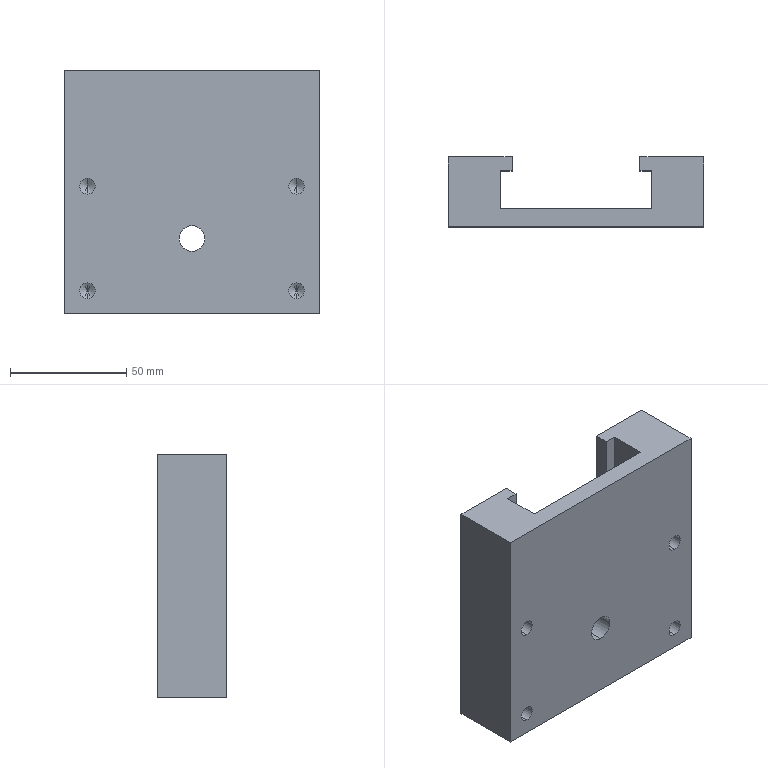Component | SolidWorks | BrassGuideRail-3 | 1 solid | 40 faces | box 110 x 30 x 105 mm | volume 198159 mm3 | cylinder 14 | plane 14 | cone 12 | commonest cylinder face diameters 6.8 x8 4.2 x4 11 x2
build123d program:
from build123d import *

# Parameters (mm, degrees)
EXTRUDE1_DEPTH        = 105
SKETCH2_R             = 5.5
EXTRUDE2_DEPTH        = 105
M5_TAPPED_HOLE1_D     = 4.2
M5_TAPPED_HOLE1_DEPTH = 14
M5_TAPPED_HOLE1_TIP   = 1.262
M8_TAPPED_HOLE2_D     = 6.8
M8_TAPPED_HOLE2_DEPTH = 22.25
M8_TAPPED_HOLE2_TIP   = 2.043


with BuildPart() as part:
    # Sketch1 → Extrude1 (new body)
    with BuildSketch(Plane.XY):
        Polygon((-55, 15), (-27.5, 15), (-27.5, 9), (-32.5, 9), (-32.5, -7), (32.5, -7), (32.5, 9), (27.5, 9), (27.5, 15), (55, 15), (55, -15), (-55, -15), align=None)
    extrude(amount=EXTRUDE1_DEPTH)

    # Sketch2 → Extrude2 (cut)
    with BuildSketch(Plane(origin=(0, -7, 0), x_dir=(1, 0, 0), z_dir=(0, 1, 0))):
        with Locations(Location((0, -32.5, 0), (0, 0, 270))):
            Circle(SKETCH2_R)
    extrude(amount=-EXTRUDE2_DEPTH, mode=Mode.SUBTRACT)

    # M5 Tapped Hole1
    with Locations(Plane(origin=(0, 15, 0), x_dir=(-1, 0, 0), z_dir=(0, 1, 0))):
        with Locations((45, 85), (-45, 85)):
            Hole(M5_TAPPED_HOLE1_D / 2, depth=M5_TAPPED_HOLE1_DEPTH)
            with Locations((0, 0, -(M5_TAPPED_HOLE1_DEPTH + M5_TAPPED_HOLE1_TIP / 2))):  # 118° drill point
                Cone(0, M5_TAPPED_HOLE1_D / 2, M5_TAPPED_HOLE1_TIP, mode=Mode.SUBTRACT)

    # M8 Tapped Hole2
    with Locations(Plane.XZ.offset(15)):
        with Locations((-45, 10), (45, 10), (45, 55), (-45, 55)):
            Hole(M8_TAPPED_HOLE2_D / 2, depth=M8_TAPPED_HOLE2_DEPTH)
            with Locations((0, 0, -(M8_TAPPED_HOLE2_DEPTH + M8_TAPPED_HOLE2_TIP / 2))):  # 118° drill point
                Cone(0, M8_TAPPED_HOLE2_D / 2, M8_TAPPED_HOLE2_TIP, mode=Mode.SUBTRACT)


solid = part.part

# Placed as in the assembly
solid = solid.moved(Location((250.216, 518.983, 27.106), (0, 0, 0)))
STEP:
#1=COLOUR_RGB('',0.7922,0.8196,0.9333);
#2=FILL_AREA_STYLE_COLOUR('',#1);
#3=FILL_AREA_STYLE('',(#2));
#4=SURFACE_STYLE_FILL_AREA(#3);
#5=SURFACE_SIDE_STYLE('',(#4));
#6=SURFACE_STYLE_USAGE(.BOTH.,#5);
#7=PRESENTATION_STYLE_ASSIGNMENT((#6));
#8=CARTESIAN_POINT('',(8.079,20.718,1.595));
#9=VERTEX_POINT('',#8);
#10=CARTESIAN_POINT('',(8.079,20.718,1.327));
#11=VERTEX_POINT('',#10);
#12=CARTESIAN_POINT('',(8.079,20.718,1.461));
#13=DIRECTION('',(0.,-1.,0.));
#14=DIRECTION('',(0.,0.,-1.));
#15=AXIS2_PLACEMENT_3D('',#12,#13,#14);
#16=CIRCLE('',#15,0.1339);
#17=EDGE_CURVE('',#9,#11,#16,.T.);
#18=ORIENTED_EDGE('',*,*,#17,.F.);
#19=CARTESIAN_POINT('',(8.079,19.842,1.595));
#20=VERTEX_POINT('',#19);
#21=CARTESIAN_POINT('',(8.079,19.842,1.595));
#22=DIRECTION('',(0.,-1.,0.));
#23=VECTOR('',#22,39.37);
#24=LINE('',#21,#23);
#25=EDGE_CURVE('',#9,#20,#24,.T.);
#26=ORIENTED_EDGE('',*,*,#25,.T.);
#27=CARTESIAN_POINT('',(8.079,19.842,1.327));
#28=VERTEX_POINT('',#27);
#29=CARTESIAN_POINT('',(8.079,19.842,1.461));
#30=DIRECTION('',(0.,-1.,0.));
#31=DIRECTION('',(0.,0.,-1.));
#32=AXIS2_PLACEMENT_3D('',#29,#30,#31);
#33=CIRCLE('',#32,0.1339);
#34=EDGE_CURVE('',#20,#28,#33,.T.);
#35=ORIENTED_EDGE('',*,*,#34,.T.);
#36=CARTESIAN_POINT('',(8.079,19.842,1.327));
#37=DIRECTION('',(0.,-1.,0.));
#38=VECTOR('',#37,39.37);
#39=LINE('',#36,#38);
#40=EDGE_CURVE('',#11,#28,#39,.T.);
#41=ORIENTED_EDGE('',*,*,#40,.F.);
#42=EDGE_LOOP('',(#18,#26,#35,#41));
#43=FACE_OUTER_BOUND('',#42,.T.);
#44=CARTESIAN_POINT('',(8.079,19.842,1.461));
#45=DIRECTION('',(0.,-1.,0.));
#46=DIRECTION('',(0.,0.,-1.));
#47=AXIS2_PLACEMENT_3D('',#44,#45,#46);
#48=CYLINDRICAL_SURFACE('',#47,0.1339);
#49=ADVANCED_FACE('',(#43),#48,.F.);
#50=CARTESIAN_POINT('',(8.079,20.798,1.461));
#51=VERTEX_POINT('',#50);
#52=CARTESIAN_POINT('',(8.079,20.718,1.327));
#53=DIRECTION('',(0.,-0.515,-0.8572));
#54=VECTOR('',#53,39.37);
#55=LINE('',#52,#54);
#56=EDGE_CURVE('',#51,#11,#55,.T.);
#57=ORIENTED_EDGE('',*,*,#56,.F.);
#58=CARTESIAN_POINT('',(8.079,20.718,1.595));
#59=DIRECTION('',(0.,-0.515,0.8572));
#60=VECTOR('',#59,39.37);
#61=LINE('',#58,#60);
#62=EDGE_CURVE('',#51,#9,#61,.T.);
#63=ORIENTED_EDGE('',*,*,#62,.T.);
#64=ORIENTED_EDGE('',*,*,#17,.T.);
#65=EDGE_LOOP('',(#57,#63,#64));
#66=FACE_OUTER_BOUND('',#65,.T.);
#67=CARTESIAN_POINT('',(8.079,20.718,1.461));
#68=DIRECTION('',(0.,-1.,0.));
#69=DIRECTION('',(0.,0.,-1.));
#70=AXIS2_PLACEMENT_3D('',#67,#68,#69);
#71=CONICAL_SURFACE('',#70,0.1339,1.03);
#72=ADVANCED_FACE('',(#66),#71,.F.);
#73=CARTESIAN_POINT('',(11.623,20.718,1.595));
#74=VERTEX_POINT('',#73);
#75=CARTESIAN_POINT('',(11.623,20.718,1.327));
#76=VERTEX_POINT('',#75);
#77=CARTESIAN_POINT('',(11.623,20.718,1.461));
#78=DIRECTION('',(0.,-1.,0.));
#79=DIRECTION('',(0.,0.,-1.));
#80=AXIS2_PLACEMENT_3D('',#77,#78,#79);
#81=CIRCLE('',#80,0.1339);
#82=EDGE_CURVE('',#74,#76,#81,.T.);
#83=ORIENTED_EDGE('',*,*,#82,.F.);
#84=CARTESIAN_POINT('',(11.623,19.842,1.595));
#85=VERTEX_POINT('',#84);
#86=CARTESIAN_POINT('',(11.623,19.842,1.595));
#87=DIRECTION('',(0.,-1.,0.));
#88=VECTOR('',#87,39.37);
#89=LINE('',#86,#88);
#90=EDGE_CURVE('',#74,#85,#89,.T.);
#91=ORIENTED_EDGE('',*,*,#90,.T.);
#92=CARTESIAN_POINT('',(11.623,19.842,1.327));
#93=VERTEX_POINT('',#92);
#94=CARTESIAN_POINT('',(11.623,19.842,1.461));
#95=DIRECTION('',(0.,-1.,0.));
#96=DIRECTION('',(0.,0.,-1.));
#97=AXIS2_PLACEMENT_3D('',#94,#95,#96);
#98=CIRCLE('',#97,0.1339);
#99=EDGE_CURVE('',#85,#93,#98,.T.);
#100=ORIENTED_EDGE('',*,*,#99,.T.);
#101=CARTESIAN_POINT('',(11.623,19.842,1.327));
#102=DIRECTION('',(0.,-1.,0.));
#103=VECTOR('',#102,39.37);
#104=LINE('',#101,#103);
#105=EDGE_CURVE('',#76,#93,#104,.T.);
#106=ORIENTED_EDGE('',*,*,#105,.F.);
#107=EDGE_LOOP('',(#83,#91,#100,#106));
#108=FACE_OUTER_BOUND('',#107,.T.);
#109=CARTESIAN_POINT('',(11.623,19.842,1.461));
#110=DIRECTION('',(0.,-1.,0.));
#111=DIRECTION('',(0.,0.,-1.));
#112=AXIS2_PLACEMENT_3D('',#109,#110,#111);
#113=CYLINDRICAL_SURFACE('',#112,0.1339);
#114=ADVANCED_FACE('',(#108),#113,.F.);
#115=CARTESIAN_POINT('',(11.623,20.798,1.461));
#116=VERTEX_POINT('',#115);
#117=CARTESIAN_POINT('',(11.623,20.718,1.327));
#118=DIRECTION('',(0.,-0.515,-0.8572));
#119=VECTOR('',#118,39.37);
#120=LINE('',#117,#119);
#121=EDGE_CURVE('',#116,#76,#120,.T.);
#122=ORIENTED_EDGE('',*,*,#121,.F.);
#123=CARTESIAN_POINT('',(11.623,20.718,1.595));
#124=DIRECTION('',(0.,-0.515,0.8572));
#125=VECTOR('',#124,39.37);
#126=LINE('',#123,#125);
#127=EDGE_CURVE('',#116,#74,#126,.T.);
#128=ORIENTED_EDGE('',*,*,#127,.T.);
#129=ORIENTED_EDGE('',*,*,#82,.T.);
#130=EDGE_LOOP('',(#122,#128,#129));
#131=FACE_OUTER_BOUND('',#130,.T.);
#132=CARTESIAN_POINT('',(11.623,20.718,1.461));
#133=DIRECTION('',(0.,-1.,0.));
#134=DIRECTION('',(0.,0.,-1.));
#135=AXIS2_PLACEMENT_3D('',#132,#133,#134);
#136=CONICAL_SURFACE('',#135,0.1339,1.03);
#137=ADVANCED_FACE('',(#131),#136,.F.);
#138=CARTESIAN_POINT('',(11.623,20.718,3.366));
#139=VERTEX_POINT('',#138);
#140=CARTESIAN_POINT('',(11.623,20.718,3.099));
#141=VERTEX_POINT('',#140);
#142=CARTESIAN_POINT('',(11.623,20.718,3.233));
#143=DIRECTION('',(0.,-1.,0.));
#144=DIRECTION('',(0.,0.,-1.));
#145=AXIS2_PLACEMENT_3D('',#142,#143,#144);
#146=CIRCLE('',#145,0.1339);
#147=EDGE_CURVE('',#139,#141,#146,.T.);
#148=ORIENTED_EDGE('',*,*,#147,.F.);
#149=CARTESIAN_POINT('',(11.623,19.842,3.366));
#150=VERTEX_POINT('',#149);
#151=CARTESIAN_POINT('',(11.623,19.842,3.366));
#152=DIRECTION('',(0.,-1.,0.));
#153=VECTOR('',#152,39.37);
#154=LINE('',#151,#153);
#155=EDGE_CURVE('',#139,#150,#154,.T.);
#156=ORIENTED_EDGE('',*,*,#155,.T.);
#157=CARTESIAN_POINT('',(11.623,19.842,3.099));
#158=VERTEX_POINT('',#157);
#159=CARTESIAN_POINT('',(11.623,19.842,3.233));
#160=DIRECTION('',(0.,-1.,0.));
#161=DIRECTION('',(0.,0.,-1.));
#162=AXIS2_PLACEMENT_3D('',#159,#160,#161);
#163=CIRCLE('',#162,0.1339);
#164=EDGE_CURVE('',#150,#158,#163,.T.);
#165=ORIENTED_EDGE('',*,*,#164,.T.);
#166=CARTESIAN_POINT('',(11.623,19.842,3.099));
#167=DIRECTION('',(0.,-1.,0.));
#168=VECTOR('',#167,39.37);
#169=LINE('',#166,#168);
#170=EDGE_CURVE('',#141,#158,#169,.T.);
#171=ORIENTED_EDGE('',*,*,#170,.F.);
#172=EDGE_LOOP('',(#148,#156,#165,#171));
#173=FACE_OUTER_BOUND('',#172,.T.);
#174=CARTESIAN_POINT('',(11.623,19.842,3.233));
#175=DIRECTION('',(0.,-1.,0.));
#176=DIRECTION('',(0.,0.,-1.));
#177=AXIS2_PLACEMENT_3D('',#174,#175,#176);
#178=CYLINDRICAL_SURFACE('',#177,0.1339);
#179=ADVANCED_FACE('',(#173),#178,.F.);
#180=CARTESIAN_POINT('',(11.623,20.798,3.233));
#181=VERTEX_POINT('',#180);
#182=CARTESIAN_POINT('',(11.623,20.718,3.099));
#183=DIRECTION('',(0.,-0.515,-0.8572));
#184=VECTOR('',#183,39.37);
#185=LINE('',#182,#184);
#186=EDGE_CURVE('',#181,#141,#185,.T.);
#187=ORIENTED_EDGE('',*,*,#186,.F.);
#188=CARTESIAN_POINT('',(11.623,20.718,3.366));
#189=DIRECTION('',(0.,-0.515,0.8572));
#190=VECTOR('',#189,39.37);
#191=LINE('',#188,#190);
#192=EDGE_CURVE('',#181,#139,#191,.T.);
#193=ORIENTED_EDGE('',*,*,#192,.T.);
#194=ORIENTED_EDGE('',*,*,#147,.T.);
#195=EDGE_LOOP('',(#187,#193,#194));
#196=FACE_OUTER_BOUND('',#195,.T.);
#197=CARTESIAN_POINT('',(11.623,20.718,3.233));
#198=DIRECTION('',(0.,-1.,0.));
#199=DIRECTION('',(0.,0.,-1.));
#200=AXIS2_PLACEMENT_3D('',#197,#198,#199);
#201=CONICAL_SURFACE('',#200,0.1339,1.03);
#202=ADVANCED_FACE('',(#196),#201,.F.);
#203=CARTESIAN_POINT('',(8.079,20.718,3.366));
#204=VERTEX_POINT('',#203);
#205=CARTESIAN_POINT('',(8.079,20.718,3.099));
#206=VERTEX_POINT('',#205);
#207=CARTESIAN_POINT('',(8.079,20.718,3.233));
#208=DIRECTION('',(0.,-1.,0.));
#209=DIRECTION('',(0.,0.,-1.));
#210=AXIS2_PLACEMENT_3D('',#207,#208,#209);
#211=CIRCLE('',#210,0.1339);
#212=EDGE_CURVE('',#204,#206,#211,.T.);
#213=ORIENTED_EDGE('',*,*,#212,.F.);
#214=CARTESIAN_POINT('',(8.079,19.842,3.366));
#215=VERTEX_POINT('',#214);
#216=CARTESIAN_POINT('',(8.079,19.842,3.366));
#217=DIRECTION('',(0.,-1.,0.));
#218=VECTOR('',#217,39.37);
#219=LINE('',#216,#218);
#220=EDGE_CURVE('',#204,#215,#219,.T.);
#221=ORIENTED_EDGE('',*,*,#220,.T.);
#222=CARTESIAN_POINT('',(8.079,19.842,3.099));
#223=VERTEX_POINT('',#222);
#224=CARTESIAN_POINT('',(8.079,19.842,3.233));
#225=DIRECTION('',(0.,-1.,0.));
#226=DIRECTION('',(0.,0.,-1.));
#227=AXIS2_PLACEMENT_3D('',#224,#225,#226);
#228=CIRCLE('',#227,0.1339);
#229=EDGE_CURVE('',#215,#223,#228,.T.);
#230=ORIENTED_EDGE('',*,*,#229,.T.);
#231=CARTESIAN_POINT('',(8.079,19.842,3.099));
#232=DIRECTION('',(0.,-1.,0.));
#233=VECTOR('',#232,39.37);
#234=LINE('',#231,#233);
#235=EDGE_CURVE('',#206,#223,#234,.T.);
#236=ORIENTED_EDGE('',*,*,#235,.F.);
#237=EDGE_LOOP('',(#213,#221,#230,#236));
#238=FACE_OUTER_BOUND('',#237,.T.);
#239=CARTESIAN_POINT('',(8.079,19.842,3.233));
#240=DIRECTION('',(0.,-1.,0.));
#241=DIRECTION('',(0.,0.,-1.));
#242=AXIS2_PLACEMENT_3D('',#239,#240,#241);
#243=CYLINDRICAL_SURFACE('',#242,0.1339);
#244=ADVANCED_FACE('',(#238),#243,.F.);
#245=CARTESIAN_POINT('',(8.079,20.798,3.233));
#246=VERTEX_POINT('',#245);
#247=CARTESIAN_POINT('',(8.079,20.718,3.099));
#248=DIRECTION('',(0.,-0.515,-0.8572));
#249=VECTOR('',#248,39.37);
#250=LINE('',#247,#249);
#251=EDGE_CURVE('',#246,#206,#250,.T.);
#252=ORIENTED_EDGE('',*,*,#251,.F.);
#253=CARTESIAN_POINT('',(8.079,20.718,3.366));
#254=DIRECTION('',(0.,-0.515,0.8572));
#255=VECTOR('',#254,39.37);
#256=LINE('',#253,#255);
#257=EDGE_CURVE('',#246,#204,#256,.T.);
#258=ORIENTED_EDGE('',*,*,#257,.T.);
#259=ORIENTED_EDGE('',*,*,#212,.T.);
#260=EDGE_LOOP('',(#252,#258,#259));
#261=FACE_OUTER_BOUND('',#260,.T.);
#262=CARTESIAN_POINT('',(8.079,20.718,3.233));
#263=DIRECTION('',(0.,-1.,0.));
#264=DIRECTION('',(0.,0.,-1.));
#265=AXIS2_PLACEMENT_3D('',#262,#263,#264);
#266=CONICAL_SURFACE('',#265,0.1339,1.03);
#267=ADVANCED_FACE('',(#261),#266,.F.);
#268=CARTESIAN_POINT('',(8.079,20.472,4.331));
#269=VERTEX_POINT('',#268);
#270=CARTESIAN_POINT('',(8.079,20.472,4.496));
#271=VERTEX_POINT('',#270);
#272=CARTESIAN_POINT('',(8.079,20.472,4.414));
#273=DIRECTION('',(0.,1.,0.));
#274=DIRECTION('',(0.,0.,1.));
#275=AXIS2_PLACEMENT_3D('',#272,#273,#274);
#276=CIRCLE('',#275,0.08268);
#277=EDGE_CURVE('',#269,#271,#276,.T.);
#278=ORIENTED_EDGE('',*,*,#277,.F.);
#279=CARTESIAN_POINT('',(8.079,21.023,4.331));
#280=VERTEX_POINT('',#279);
#281=CARTESIAN_POINT('',(8.079,21.023,4.331));
#282=DIRECTION('',(0.,1.,0.));
#283=VECTOR('',#282,39.37);
#284=LINE('',#281,#283);
#285=EDGE_CURVE('',#269,#280,#284,.T.);
#286=ORIENTED_EDGE('',*,*,#285,.T.);
#287=CARTESIAN_POINT('',(8.079,21.023,4.496));
#288=VERTEX_POINT('',#287);
#289=CARTESIAN_POINT('',(8.079,21.023,4.414));
#290=DIRECTION('',(0.,1.,0.));
#291=DIRECTION('',(0.,0.,1.));
#292=AXIS2_PLACEMENT_3D('',#289,#290,#291);
#293=CIRCLE('',#292,0.08268);
#294=EDGE_CURVE('',#280,#288,#293,.T.);
#295=ORIENTED_EDGE('',*,*,#294,.T.);
#296=CARTESIAN_POINT('',(8.079,21.023,4.496));
#297=DIRECTION('',(0.,1.,0.));
#298=VECTOR('',#297,39.37);
#299=LINE('',#296,#298);
#300=EDGE_CURVE('',#271,#288,#299,.T.);
#301=ORIENTED_EDGE('',*,*,#300,.F.);
#302=EDGE_LOOP('',(#278,#286,#295,#301));
#303=FACE_OUTER_BOUND('',#302,.T.);
#304=CARTESIAN_POINT('',(8.079,21.023,4.414));
#305=DIRECTION('',(0.,1.,0.));
#306=DIRECTION('',(0.,0.,1.));
#307=AXIS2_PLACEMENT_3D('',#304,#305,#306);
#308=CYLINDRICAL_SURFACE('',#307,0.08268);
#309=ADVANCED_FACE('',(#303),#308,.F.);
#310=CARTESIAN_POINT('',(8.079,20.422,4.414));
#311=VERTEX_POINT('',#310);
#312=CARTESIAN_POINT('',(8.079,20.472,4.496));
#313=DIRECTION('',(0.,0.515,0.8572));
#314=VECTOR('',#313,39.37);
#315=LINE('',#312,#314);
#316=EDGE_CURVE('',#311,#271,#315,.T.);
#317=ORIENTED_EDGE('',*,*,#316,.F.);
#318=CARTESIAN_POINT('',(8.079,20.472,4.331));
#319=DIRECTION('',(0.,0.515,-0.8572));
#320=VECTOR('',#319,39.37);
#321=LINE('',#318,#320);
#322=EDGE_CURVE('',#311,#269,#321,.T.);
#323=ORIENTED_EDGE('',*,*,#322,.T.);
#324=ORIENTED_EDGE('',*,*,#277,.T.);
#325=EDGE_LOOP('',(#317,#323,#324));
#326=FACE_OUTER_BOUND('',#325,.T.);
#327=CARTESIAN_POINT('',(8.079,20.472,4.414));
#328=DIRECTION('',(0.,1.,0.));
#329=DIRECTION('',(0.,0.,1.));
#330=AXIS2_PLACEMENT_3D('',#327,#328,#329);
#331=CONICAL_SURFACE('',#330,0.08268,1.03);
#332=ADVANCED_FACE('',(#326),#331,.F.);
#333=CARTESIAN_POINT('',(11.623,20.472,4.331));
#334=VERTEX_POINT('',#333);
#335=CARTESIAN_POINT('',(11.623,20.472,4.496));
#336=VERTEX_POINT('',#335);
#337=CARTESIAN_POINT('',(11.623,20.472,4.414));
#338=DIRECTION('',(0.,1.,0.));
#339=DIRECTION('',(0.,0.,1.));
#340=AXIS2_PLACEMENT_3D('',#337,#338,#339);
#341=CIRCLE('',#340,0.08268);
#342=EDGE_CURVE('',#334,#336,#341,.T.);
#343=ORIENTED_EDGE('',*,*,#342,.F.);
#344=CARTESIAN_POINT('',(11.623,21.023,4.331));
#345=VERTEX_POINT('',#344);
#346=CARTESIAN_POINT('',(11.623,21.023,4.331));
#347=DIRECTION('',(0.,1.,0.));
#348=VECTOR('',#347,39.37);
#349=LINE('',#346,#348);
#350=EDGE_CURVE('',#334,#345,#349,.T.);
#351=ORIENTED_EDGE('',*,*,#350,.T.);
#352=CARTESIAN_POINT('',(11.623,21.023,4.496));
#353=VERTEX_POINT('',#352);
#354=CARTESIAN_POINT('',(11.623,21.023,4.414));
#355=DIRECTION('',(0.,1.,0.));
#356=DIRECTION('',(0.,0.,1.));
#357=AXIS2_PLACEMENT_3D('',#354,#355,#356);
#358=CIRCLE('',#357,0.08268);
#359=EDGE_CURVE('',#345,#353,#358,.T.);
#360=ORIENTED_EDGE('',*,*,#359,.T.);
#361=CARTESIAN_POINT('',(11.623,21.023,4.496));
#362=DIRECTION('',(0.,1.,0.));
#363=VECTOR('',#362,39.37);
#364=LINE('',#361,#363);
#365=EDGE_CURVE('',#336,#353,#364,.T.);
#366=ORIENTED_EDGE('',*,*,#365,.F.);
#367=EDGE_LOOP('',(#343,#351,#360,#366));
#368=FACE_OUTER_BOUND('',#367,.T.);
#369=CARTESIAN_POINT('',(11.623,21.023,4.414));
#370=DIRECTION('',(0.,1.,0.));
#371=DIRECTION('',(0.,0.,1.));
#372=AXIS2_PLACEMENT_3D('',#369,#370,#371);
#373=CYLINDRICAL_SURFACE('',#372,0.08268);
#374=ADVANCED_FACE('',(#368),#373,.F.);
#375=CARTESIAN_POINT('',(11.623,20.422,4.414));
#376=VERTEX_POINT('',#375);
#377=CARTESIAN_POINT('',(11.623,20.472,4.496));
#378=DIRECTION('',(0.,0.515,0.8572));
#379=VECTOR('',#378,39.37);
#380=LINE('',#377,#379);
#381=EDGE_CURVE('',#376,#336,#380,.T.);
#382=ORIENTED_EDGE('',*,*,#381,.F.);
#383=CARTESIAN_POINT('',(11.623,20.472,4.331));
#384=DIRECTION('',(0.,0.515,-0.8572));
#385=VECTOR('',#384,39.37);
#386=LINE('',#383,#385);
#387=EDGE_CURVE('',#376,#334,#386,.T.);
#388=ORIENTED_EDGE('',*,*,#387,.T.);
#389=ORIENTED_EDGE('',*,*,#342,.T.);
#390=EDGE_LOOP('',(#382,#388,#389));
#391=FACE_OUTER_BOUND('',#390,.T.);
#392=CARTESIAN_POINT('',(11.623,20.472,4.414));
#393=DIRECTION('',(0.,1.,0.));
#394=DIRECTION('',(0.,0.,1.));
#395=AXIS2_PLACEMENT_3D('',#392,#393,#394);
#396=CONICAL_SURFACE('',#395,0.08268,1.03);
#397=ADVANCED_FACE('',(#391),#396,.F.);
#398=CARTESIAN_POINT('',(9.851,19.842,2.13));
#399=VERTEX_POINT('',#398);
#400=CARTESIAN_POINT('',(9.851,19.842,2.563));
#401=VERTEX_POINT('',#400);
#402=CARTESIAN_POINT('',(9.851,19.842,2.347));
#403=DIRECTION('',(0.,1.,0.));
#404=DIRECTION('',(0.,0.,1.));
#405=AXIS2_PLACEMENT_3D('',#402,#403,#404);
#406=CIRCLE('',#405,0.2165);
#407=EDGE_CURVE('',#399,#401,#406,.T.);
#408=ORIENTED_EDGE('',*,*,#407,.F.);
#409=CARTESIAN_POINT('',(9.851,20.157,2.13));
#410=VERTEX_POINT('',#409);
#411=CARTESIAN_POINT('',(9.851,16.023,2.13));
#412=DIRECTION('',(0.,1.,0.));
#413=VECTOR('',#412,39.37);
#414=LINE('',#411,#413);
#415=EDGE_CURVE('',#399,#410,#414,.T.);
#416=ORIENTED_EDGE('',*,*,#415,.T.);
#417=CARTESIAN_POINT('',(9.851,20.157,2.563));
#418=VERTEX_POINT('',#417);
#419=CARTESIAN_POINT('',(9.851,20.157,2.347));
#420=DIRECTION('',(0.,1.,0.));
#421=DIRECTION('',(0.,0.,1.));
#422=AXIS2_PLACEMENT_3D('',#419,#420,#421);
#423=CIRCLE('',#422,0.2165);
#424=EDGE_CURVE('',#410,#418,#423,.T.);
#425=ORIENTED_EDGE('',*,*,#424,.T.);
#426=CARTESIAN_POINT('',(9.851,16.023,2.563));
#427=DIRECTION('',(0.,1.,0.));
#428=VECTOR('',#427,39.37);
#429=LINE('',#426,#428);
#430=EDGE_CURVE('',#401,#418,#429,.T.);
#431=ORIENTED_EDGE('',*,*,#430,.F.);
#432=EDGE_LOOP('',(#408,#416,#425,#431));
#433=FACE_OUTER_BOUND('',#432,.T.);
#434=CARTESIAN_POINT('',(9.851,16.023,2.347));
#435=DIRECTION('',(0.,1.,0.));
#436=DIRECTION('',(0.,0.,1.));
#437=AXIS2_PLACEMENT_3D('',#434,#435,#436);
#438=CYLINDRICAL_SURFACE('',#437,0.2165);
#439=ADVANCED_FACE('',(#433),#438,.F.);
#440=CARTESIAN_POINT('',(7.686,21.023,1.067));
#441=VERTEX_POINT('',#440);
#442=CARTESIAN_POINT('',(7.686,19.842,1.067));
#443=VERTEX_POINT('',#442);
#444=CARTESIAN_POINT('',(7.686,21.023,1.067));
#445=DIRECTION('',(0.,-1.,0.));
#446=VECTOR('',#445,39.37);
#447=LINE('',#444,#446);
#448=EDGE_CURVE('',#441,#443,#447,.T.);
#449=ORIENTED_EDGE('',*,*,#448,.T.);
#450=CARTESIAN_POINT('',(7.686,19.842,5.201));
#451=VERTEX_POINT('',#450);
#452=CARTESIAN_POINT('',(7.686,19.842,5.201));
#453=DIRECTION('',(0.,0.,-1.));
#454=VECTOR('',#453,39.37);
#455=LINE('',#452,#454);
#456=EDGE_CURVE('',#451,#443,#455,.T.);
#457=ORIENTED_EDGE('',*,*,#456,.F.);
#458=CARTESIAN_POINT('',(7.686,21.023,5.201));
#459=VERTEX_POINT('',#458);
#460=CARTESIAN_POINT('',(7.686,21.023,5.201));
#461=DIRECTION('',(0.,-1.,0.));
#462=VECTOR('',#461,39.37);
#463=LINE('',#460,#462);
#464=EDGE_CURVE('',#459,#451,#463,.T.);
#465=ORIENTED_EDGE('',*,*,#464,.F.);
#466=CARTESIAN_POINT('',(7.686,21.023,5.201));
#467=DIRECTION('',(0.,0.,-1.));
#468=VECTOR('',#467,39.37);
#469=LINE('',#466,#468);
#470=EDGE_CURVE('',#459,#441,#469,.T.);
#471=ORIENTED_EDGE('',*,*,#470,.T.);
#472=EDGE_LOOP('',(#449,#457,#465,#471));
#473=FACE_OUTER_BOUND('',#472,.T.);
#474=CARTESIAN_POINT('',(7.686,21.023,5.201));
#475=DIRECTION('',(1.,0.,0.));
#476=DIRECTION('',(0.,0.,-1.));
#477=AXIS2_PLACEMENT_3D('',#474,#475,#476);
#478=PLANE('',#477);
#479=ADVANCED_FACE('',(#473),#478,.F.);
#480=CARTESIAN_POINT('',(8.079,19.842,1.461));
#481=DIRECTION('',(0.,-1.,0.));
#482=DIRECTION('',(0.,0.,-1.));
#483=AXIS2_PLACEMENT_3D('',#480,#481,#482);
#484=CIRCLE('',#483,0.1339);
#485=EDGE_CURVE('',#28,#20,#484,.T.);
#486=ORIENTED_EDGE('',*,*,#485,.F.);
#487=ORIENTED_EDGE('',*,*,#34,.F.);
#488=EDGE_LOOP('',(#486,#487));
#489=FACE_BOUND('',#488,.T.);
#490=CARTESIAN_POINT('',(11.623,19.842,1.461));
#491=DIRECTION('',(0.,-1.,0.));
#492=DIRECTION('',(0.,0.,-1.));
#493=AXIS2_PLACEMENT_3D('',#490,#491,#492);
#494=CIRCLE('',#493,0.1339);
#495=EDGE_CURVE('',#93,#85,#494,.T.);
#496=ORIENTED_EDGE('',*,*,#495,.F.);
#497=ORIENTED_EDGE('',*,*,#99,.F.);
#498=EDGE_LOOP('',(#496,#497));
#499=FACE_BOUND('',#498,.T.);
#500=CARTESIAN_POINT('',(11.623,19.842,3.233));
#501=DIRECTION('',(0.,-1.,0.));
#502=DIRECTION('',(0.,0.,-1.));
#503=AXIS2_PLACEMENT_3D('',#500,#501,#502);
#504=CIRCLE('',#503,0.1339);
#505=EDGE_CURVE('',#158,#150,#504,.T.);
#506=ORIENTED_EDGE('',*,*,#505,.F.);
#507=ORIENTED_EDGE('',*,*,#164,.F.);
#508=EDGE_LOOP('',(#506,#507));
#509=FACE_BOUND('',#508,.T.);
#510=CARTESIAN_POINT('',(8.079,19.842,3.233));
#511=DIRECTION('',(0.,-1.,0.));
#512=DIRECTION('',(0.,0.,-1.));
#513=AXIS2_PLACEMENT_3D('',#510,#511,#512);
#514=CIRCLE('',#513,0.1339);
#515=EDGE_CURVE('',#223,#215,#514,.T.);
#516=ORIENTED_EDGE('',*,*,#515,.F.);
#517=ORIENTED_EDGE('',*,*,#229,.F.);
#518=EDGE_LOOP('',(#516,#517));
#519=FACE_BOUND('',#518,.T.);
#520=CARTESIAN_POINT('',(9.851,19.842,2.347));
#521=DIRECTION('',(0.,1.,0.));
#522=DIRECTION('',(0.,0.,1.));
#523=AXIS2_PLACEMENT_3D('',#520,#521,#522);
#524=CIRCLE('',#523,0.2165);
#525=EDGE_CURVE('',#401,#399,#524,.T.);
#526=ORIENTED_EDGE('',*,*,#525,.T.);
#527=ORIENTED_EDGE('',*,*,#407,.T.);
#528=EDGE_LOOP('',(#526,#527));
#529=FACE_BOUND('',#528,.T.);
#530=CARTESIAN_POINT('',(12.016,19.842,1.067));
#531=VERTEX_POINT('',#530);
#532=CARTESIAN_POINT('',(7.686,19.842,1.067));
#533=DIRECTION('',(1.,0.,0.));
#534=VECTOR('',#533,39.37);
#535=LINE('',#532,#534);
#536=EDGE_CURVE('',#443,#531,#535,.T.);
#537=ORIENTED_EDGE('',*,*,#536,.T.);
#538=CARTESIAN_POINT('',(12.016,19.842,5.201));
#539=VERTEX_POINT('',#538);
#540=CARTESIAN_POINT('',(12.016,19.842,5.201));
#541=DIRECTION('',(0.,0.,-1.));
#542=VECTOR('',#541,39.37);
#543=LINE('',#540,#542);
#544=EDGE_CURVE('',#539,#531,#543,.T.);
#545=ORIENTED_EDGE('',*,*,#544,.F.);
#546=CARTESIAN_POINT('',(7.686,19.842,5.201));
#547=DIRECTION('',(1.,0.,0.));
#548=VECTOR('',#547,39.37);
#549=LINE('',#546,#548);
#550=EDGE_CURVE('',#451,#539,#549,.T.);
#551=ORIENTED_EDGE('',*,*,#550,.F.);
#552=ORIENTED_EDGE('',*,*,#456,.T.);
#553=EDGE_LOOP('',(#537,#545,#551,#552));
#554=FACE_OUTER_BOUND('',#553,.T.);
#555=CARTESIAN_POINT('',(7.686,19.842,5.201));
#556=DIRECTION('',(0.,1.,0.));
#557=DIRECTION('',(0.,0.,1.));
#558=AXIS2_PLACEMENT_3D('',#555,#556,#557);
#559=PLANE('',#558);
#560=ADVANCED_FACE('',(#489,#499,#509,#519,#529,#554),#559,.F.);
#561=CARTESIAN_POINT('',(12.016,21.023,1.067));
#562=VERTEX_POINT('',#561);
#563=CARTESIAN_POINT('',(12.016,21.023,1.067));
#564=DIRECTION('',(0.,1.,0.));
#565=VECTOR('',#564,39.37);
#566=LINE('',#563,#565);
#567=EDGE_CURVE('',#531,#562,#566,.T.);
#568=ORIENTED_EDGE('',*,*,#567,.T.);
#569=CARTESIAN_POINT('',(12.016,21.023,5.201));
#570=VERTEX_POINT('',#569);
#571=CARTESIAN_POINT('',(12.016,21.023,5.201));
#572=DIRECTION('',(0.,0.,-1.));
#573=VECTOR('',#572,39.37);
#574=LINE('',#571,#573);
#575=EDGE_CURVE('',#570,#562,#574,.T.);
#576=ORIENTED_EDGE('',*,*,#575,.F.);
#577=CARTESIAN_POINT('',(12.016,21.023,5.201));
#578=DIRECTION('',(0.,1.,0.));
#579=VECTOR('',#578,39.37);
#580=LINE('',#577,#579);
#581=EDGE_CURVE('',#539,#570,#580,.T.);
#582=ORIENTED_EDGE('',*,*,#581,.F.);
#583=ORIENTED_EDGE('',*,*,#544,.T.);
#584=EDGE_LOOP('',(#568,#576,#582,#583));
#585=FACE_OUTER_BOUND('',#584,.T.);
#586=CARTESIAN_POINT('',(12.016,21.023,5.201));
#587=DIRECTION('',(-1.,0.,0.));
#588=DIRECTION('',(0.,0.,1.));
#589=AXIS2_PLACEMENT_3D('',#586,#587,#588);
#590=PLANE('',#589);
#591=ADVANCED_FACE('',(#585),#590,.F.);
#592=CARTESIAN_POINT('',(11.623,21.023,4.414));
#593=DIRECTION('',(0.,1.,0.));
#594=DIRECTION('',(0.,0.,1.));
#595=AXIS2_PLACEMENT_3D('',#592,#593,#594);
#596=CIRCLE('',#595,0.08268);
#597=EDGE_CURVE('',#353,#345,#596,.T.);
#598=ORIENTED_EDGE('',*,*,#597,.F.);
#599=ORIENTED_EDGE('',*,*,#359,.F.);
#600=EDGE_LOOP('',(#598,#599));
#601=FACE_BOUND('',#600,.T.);
#602=CARTESIAN_POINT('',(10.934,21.023,1.067));
#603=VERTEX_POINT('',#602);
#604=CARTESIAN_POINT('',(10.934,21.023,1.067));
#605=DIRECTION('',(-1.,0.,0.));
#606=VECTOR('',#605,39.37);
#607=LINE('',#604,#606);
#608=EDGE_CURVE('',#562,#603,#607,.T.);
#609=ORIENTED_EDGE('',*,*,#608,.T.);
#610=CARTESIAN_POINT('',(10.934,21.023,5.201));
#611=VERTEX_POINT('',#610);
#612=CARTESIAN_POINT('',(10.934,21.023,5.201));
#613=DIRECTION('',(0.,0.,-1.));
#614=VECTOR('',#613,39.37);
#615=LINE('',#612,#614);
#616=EDGE_CURVE('',#611,#603,#615,.T.);
#617=ORIENTED_EDGE('',*,*,#616,.F.);
#618=CARTESIAN_POINT('',(10.934,21.023,5.201));
#619=DIRECTION('',(-1.,0.,0.));
#620=VECTOR('',#619,39.37);
#621=LINE('',#618,#620);
#622=EDGE_CURVE('',#570,#611,#621,.T.);
#623=ORIENTED_EDGE('',*,*,#622,.F.);
#624=ORIENTED_EDGE('',*,*,#575,.T.);
#625=EDGE_LOOP('',(#609,#617,#623,#624));
#626=FACE_OUTER_BOUND('',#625,.T.);
#627=CARTESIAN_POINT('',(10.934,21.023,5.201));
#628=DIRECTION('',(0.,-1.,0.));
#629=DIRECTION('',(0.,0.,-1.));
#630=AXIS2_PLACEMENT_3D('',#627,#628,#629);
#631=PLANE('',#630);
#632=ADVANCED_FACE('',(#601,#626),#631,.F.);
#633=CARTESIAN_POINT('',(10.934,20.787,1.067));
#634=VERTEX_POINT('',#633);
#635=CARTESIAN_POINT('',(10.934,21.023,1.067));
#636=DIRECTION('',(0.,-1.,0.));
#637=VECTOR('',#636,39.37);
#638=LINE('',#635,#637);
#639=EDGE_CURVE('',#603,#634,#638,.T.);
#640=ORIENTED_EDGE('',*,*,#639,.T.);
#641=CARTESIAN_POINT('',(10.934,20.787,5.201));
#642=VERTEX_POINT('',#641);
#643=CARTESIAN_POINT('',(10.934,20.787,5.201));
#644=DIRECTION('',(0.,0.,-1.));
#645=VECTOR('',#644,39.37);
#646=LINE('',#643,#645);
#647=EDGE_CURVE('',#642,#634,#646,.T.);
#648=ORIENTED_EDGE('',*,*,#647,.F.);
#649=CARTESIAN_POINT('',(10.934,21.023,5.201));
#650=DIRECTION('',(0.,-1.,0.));
#651=VECTOR('',#650,39.37);
#652=LINE('',#649,#651);
#653=EDGE_CURVE('',#611,#642,#652,.T.);
#654=ORIENTED_EDGE('',*,*,#653,.F.);
#655=ORIENTED_EDGE('',*,*,#616,.T.);
#656=EDGE_LOOP('',(#640,#648,#654,#655));
#657=FACE_OUTER_BOUND('',#656,.T.);
#658=CARTESIAN_POINT('',(10.934,21.023,5.201));
#659=DIRECTION('',(1.,0.,0.));
#660=DIRECTION('',(0.,0.,-1.));
#661=AXIS2_PLACEMENT_3D('',#658,#659,#660);
#662=PLANE('',#661);
#663=ADVANCED_FACE('',(#657),#662,.F.);
#664=CARTESIAN_POINT('',(11.131,20.787,1.067));
#665=VERTEX_POINT('',#664);
#666=CARTESIAN_POINT('',(10.934,20.787,1.067));
#667=DIRECTION('',(1.,0.,0.));
#668=VECTOR('',#667,39.37);
#669=LINE('',#666,#668);
#670=EDGE_CURVE('',#634,#665,#669,.T.);
#671=ORIENTED_EDGE('',*,*,#670,.T.);
#672=CARTESIAN_POINT('',(11.131,20.787,5.201));
#673=VERTEX_POINT('',#672);
#674=CARTESIAN_POINT('',(11.131,20.787,5.201));
#675=DIRECTION('',(0.,0.,-1.));
#676=VECTOR('',#675,39.37);
#677=LINE('',#674,#676);
#678=EDGE_CURVE('',#673,#665,#677,.T.);
#679=ORIENTED_EDGE('',*,*,#678,.F.);
#680=CARTESIAN_POINT('',(10.934,20.787,5.201));
#681=DIRECTION('',(1.,0.,0.));
#682=VECTOR('',#681,39.37);
#683=LINE('',#680,#682);
#684=EDGE_CURVE('',#642,#673,#683,.T.);
#685=ORIENTED_EDGE('',*,*,#684,.F.);
#686=ORIENTED_EDGE('',*,*,#647,.T.);
#687=EDGE_LOOP('',(#671,#679,#685,#686));
#688=FACE_OUTER_BOUND('',#687,.T.);
#689=CARTESIAN_POINT('',(10.934,20.787,5.201));
#690=DIRECTION('',(0.,1.,0.));
#691=DIRECTION('',(0.,0.,1.));
#692=AXIS2_PLACEMENT_3D('',#689,#690,#691);
#693=PLANE('',#692);
#694=ADVANCED_FACE('',(#688),#693,.F.);
#695=CARTESIAN_POINT('',(11.131,20.157,1.067));
#696=VERTEX_POINT('',#695);
#697=CARTESIAN_POINT('',(11.131,20.787,1.067));
#698=DIRECTION('',(0.,-1.,0.));
#699=VECTOR('',#698,39.37);
#700=LINE('',#697,#699);
#701=EDGE_CURVE('',#665,#696,#700,.T.);
#702=ORIENTED_EDGE('',*,*,#701,.T.);
#703=CARTESIAN_POINT('',(11.131,20.157,5.201));
#704=VERTEX_POINT('',#703);
#705=CARTESIAN_POINT('',(11.131,20.157,5.201));
#706=DIRECTION('',(0.,0.,-1.));
#707=VECTOR('',#706,39.37);
#708=LINE('',#705,#707);
#709=EDGE_CURVE('',#704,#696,#708,.T.);
#710=ORIENTED_EDGE('',*,*,#709,.F.);
#711=CARTESIAN_POINT('',(11.131,20.787,5.201));
#712=DIRECTION('',(0.,-1.,0.));
#713=VECTOR('',#712,39.37);
#714=LINE('',#711,#713);
#715=EDGE_CURVE('',#673,#704,#714,.T.);
#716=ORIENTED_EDGE('',*,*,#715,.F.);
#717=ORIENTED_EDGE('',*,*,#678,.T.);
#718=EDGE_LOOP('',(#702,#710,#716,#717));
#719=FACE_OUTER_BOUND('',#718,.T.);
#720=CARTESIAN_POINT('',(11.131,20.787,5.201));
#721=DIRECTION('',(1.,0.,0.));
#722=DIRECTION('',(0.,0.,-1.));
#723=AXIS2_PLACEMENT_3D('',#720,#721,#722);
#724=PLANE('',#723);
#725=ADVANCED_FACE('',(#719),#724,.F.);
#726=CARTESIAN_POINT('',(9.851,20.157,2.347));
#727=DIRECTION('',(0.,1.,0.));
#728=DIRECTION('',(0.,0.,1.));
#729=AXIS2_PLACEMENT_3D('',#726,#727,#728);
#730=CIRCLE('',#729,0.2165);
#731=EDGE_CURVE('',#418,#410,#730,.T.);
#732=ORIENTED_EDGE('',*,*,#731,.F.);
#733=ORIENTED_EDGE('',*,*,#424,.F.);
#734=EDGE_LOOP('',(#732,#733));
#735=FACE_BOUND('',#734,.T.);
#736=CARTESIAN_POINT('',(8.572,20.157,1.067));
#737=VERTEX_POINT('',#736);
#738=CARTESIAN_POINT('',(8.572,20.157,1.067));
#739=DIRECTION('',(-1.,0.,0.));
#740=VECTOR('',#739,39.37);
#741=LINE('',#738,#740);
#742=EDGE_CURVE('',#696,#737,#741,.T.);
#743=ORIENTED_EDGE('',*,*,#742,.T.);
#744=CARTESIAN_POINT('',(8.572,20.157,5.201));
#745=VERTEX_POINT('',#744);
#746=CARTESIAN_POINT('',(8.572,20.157,5.201));
#747=DIRECTION('',(0.,0.,-1.));
#748=VECTOR('',#747,39.37);
#749=LINE('',#746,#748);
#750=EDGE_CURVE('',#745,#737,#749,.T.);
#751=ORIENTED_EDGE('',*,*,#750,.F.);
#752=CARTESIAN_POINT('',(8.572,20.157,5.201));
#753=DIRECTION('',(-1.,0.,0.));
#754=VECTOR('',#753,39.37);
#755=LINE('',#752,#754);
#756=EDGE_CURVE('',#704,#745,#755,.T.);
#757=ORIENTED_EDGE('',*,*,#756,.F.);
#758=ORIENTED_EDGE('',*,*,#709,.T.);
#759=EDGE_LOOP('',(#743,#751,#757,#758));
#760=FACE_OUTER_BOUND('',#759,.T.);
#761=CARTESIAN_POINT('',(8.572,20.157,5.201));
#762=DIRECTION('',(0.,-1.,0.));
#763=DIRECTION('',(0.,0.,-1.));
#764=AXIS2_PLACEMENT_3D('',#761,#762,#763);
#765=PLANE('',#764);
#766=ADVANCED_FACE('',(#735,#760),#765,.F.);
#767=CARTESIAN_POINT('',(8.572,20.787,1.067));
#768=VERTEX_POINT('',#767);
#769=CARTESIAN_POINT('',(8.572,20.787,1.067));
#770=DIRECTION('',(0.,1.,0.));
#771=VECTOR('',#770,39.37);
#772=LINE('',#769,#771);
#773=EDGE_CURVE('',#737,#768,#772,.T.);
#774=ORIENTED_EDGE('',*,*,#773,.T.);
#775=CARTESIAN_POINT('',(8.572,20.787,5.201));
#776=VERTEX_POINT('',#775);
#777=CARTESIAN_POINT('',(8.572,20.787,5.201));
#778=DIRECTION('',(0.,0.,-1.));
#779=VECTOR('',#778,39.37);
#780=LINE('',#777,#779);
#781=EDGE_CURVE('',#776,#768,#780,.T.);
#782=ORIENTED_EDGE('',*,*,#781,.F.);
#783=CARTESIAN_POINT('',(8.572,20.787,5.201));
#784=DIRECTION('',(0.,1.,0.));
#785=VECTOR('',#784,39.37);
#786=LINE('',#783,#785);
#787=EDGE_CURVE('',#745,#776,#786,.T.);
#788=ORIENTED_EDGE('',*,*,#787,.F.);
#789=ORIENTED_EDGE('',*,*,#750,.T.);
#790=EDGE_LOOP('',(#774,#782,#788,#789));
#791=FACE_OUTER_BOUND('',#790,.T.);
#792=CARTESIAN_POINT('',(8.572,20.787,5.201));
#793=DIRECTION('',(-1.,0.,0.));
#794=DIRECTION('',(0.,0.,1.));
#795=AXIS2_PLACEMENT_3D('',#792,#793,#794);
#796=PLANE('',#795);
#797=ADVANCED_FACE('',(#791),#796,.F.);
#798=CARTESIAN_POINT('',(8.768,20.787,1.067));
#799=VERTEX_POINT('',#798);
#800=CARTESIAN_POINT('',(8.768,20.787,1.067));
#801=DIRECTION('',(1.,0.,0.));
#802=VECTOR('',#801,39.37);
#803=LINE('',#800,#802);
#804=EDGE_CURVE('',#768,#799,#803,.T.);
#805=ORIENTED_EDGE('',*,*,#804,.T.);
#806=CARTESIAN_POINT('',(8.768,20.787,5.201));
#807=VERTEX_POINT('',#806);
#808=CARTESIAN_POINT('',(8.768,20.787,5.201));
#809=DIRECTION('',(0.,0.,-1.));
#810=VECTOR('',#809,39.37);
#811=LINE('',#808,#810);
#812=EDGE_CURVE('',#807,#799,#811,.T.);
#813=ORIENTED_EDGE('',*,*,#812,.F.);
#814=CARTESIAN_POINT('',(8.768,20.787,5.201));
#815=DIRECTION('',(1.,0.,0.));
#816=VECTOR('',#815,39.37);
#817=LINE('',#814,#816);
#818=EDGE_CURVE('',#776,#807,#817,.T.);
#819=ORIENTED_EDGE('',*,*,#818,.F.);
#820=ORIENTED_EDGE('',*,*,#781,.T.);
#821=EDGE_LOOP('',(#805,#813,#819,#820));
#822=FACE_OUTER_BOUND('',#821,.T.);
#823=CARTESIAN_POINT('',(8.768,20.787,5.201));
#824=DIRECTION('',(0.,1.,0.));
#825=DIRECTION('',(0.,0.,1.));
#826=AXIS2_PLACEMENT_3D('',#823,#824,#825);
#827=PLANE('',#826);
#828=ADVANCED_FACE('',(#822),#827,.F.);
#829=CARTESIAN_POINT('',(8.768,21.023,1.067));
#830=VERTEX_POINT('',#829);
#831=CARTESIAN_POINT('',(8.768,21.023,1.067));
#832=DIRECTION('',(0.,1.,0.));
#833=VECTOR('',#832,39.37);
#834=LINE('',#831,#833);
#835=EDGE_CURVE('',#799,#830,#834,.T.);
#836=ORIENTED_EDGE('',*,*,#835,.T.);
#837=CARTESIAN_POINT('',(8.768,21.023,5.201));
#838=VERTEX_POINT('',#837);
#839=CARTESIAN_POINT('',(8.768,21.023,5.201));
#840=DIRECTION('',(0.,0.,-1.));
#841=VECTOR('',#840,39.37);
#842=LINE('',#839,#841);
#843=EDGE_CURVE('',#838,#830,#842,.T.);
#844=ORIENTED_EDGE('',*,*,#843,.F.);
#845=CARTESIAN_POINT('',(8.768,21.023,5.201));
#846=DIRECTION('',(0.,1.,0.));
#847=VECTOR('',#846,39.37);
#848=LINE('',#845,#847);
#849=EDGE_CURVE('',#807,#838,#848,.T.);
#850=ORIENTED_EDGE('',*,*,#849,.F.);
#851=ORIENTED_EDGE('',*,*,#812,.T.);
#852=EDGE_LOOP('',(#836,#844,#850,#851));
#853=FACE_OUTER_BOUND('',#852,.T.);
#854=CARTESIAN_POINT('',(8.768,21.023,5.201));
#855=DIRECTION('',(-1.,0.,0.));
#856=DIRECTION('',(0.,0.,1.));
#857=AXIS2_PLACEMENT_3D('',#854,#855,#856);
#858=PLANE('',#857);
#859=ADVANCED_FACE('',(#853),#858,.F.);
#860=CARTESIAN_POINT('',(8.079,21.023,4.414));
#861=DIRECTION('',(0.,1.,0.));
#862=DIRECTION('',(0.,0.,1.));
#863=AXIS2_PLACEMENT_3D('',#860,#861,#862);
#864=CIRCLE('',#863,0.08268);
#865=EDGE_CURVE('',#288,#280,#864,.T.);
#866=ORIENTED_EDGE('',*,*,#865,.F.);
#867=ORIENTED_EDGE('',*,*,#294,.F.);
#868=EDGE_LOOP('',(#866,#867));
#869=FACE_BOUND('',#868,.T.);
#870=CARTESIAN_POINT('',(7.686,21.023,1.067));
#871=DIRECTION('',(-1.,0.,0.));
#872=VECTOR('',#871,39.37);
#873=LINE('',#870,#872);
#874=EDGE_CURVE('',#830,#441,#873,.T.);
#875=ORIENTED_EDGE('',*,*,#874,.T.);
#876=ORIENTED_EDGE('',*,*,#470,.F.);
#877=CARTESIAN_POINT('',(7.686,21.023,5.201));
#878=DIRECTION('',(-1.,0.,0.));
#879=VECTOR('',#878,39.37);
#880=LINE('',#877,#879);
#881=EDGE_CURVE('',#838,#459,#880,.T.);
#882=ORIENTED_EDGE('',*,*,#881,.F.);
#883=ORIENTED_EDGE('',*,*,#843,.T.);
#884=EDGE_LOOP('',(#875,#876,#882,#883));
#885=FACE_OUTER_BOUND('',#884,.T.);
#886=CARTESIAN_POINT('',(7.686,21.023,5.201));
#887=DIRECTION('',(0.,-1.,0.));
#888=DIRECTION('',(0.,0.,-1.));
#889=AXIS2_PLACEMENT_3D('',#886,#887,#888);
#890=PLANE('',#889);
#891=ADVANCED_FACE('',(#869,#885),#890,.F.);
#892=ORIENTED_EDGE('',*,*,#464,.T.);
#893=ORIENTED_EDGE('',*,*,#550,.T.);
#894=ORIENTED_EDGE('',*,*,#581,.T.);
#895=ORIENTED_EDGE('',*,*,#622,.T.);
#896=ORIENTED_EDGE('',*,*,#653,.T.);
#897=ORIENTED_EDGE('',*,*,#684,.T.);
#898=ORIENTED_EDGE('',*,*,#715,.T.);
#899=ORIENTED_EDGE('',*,*,#756,.T.);
#900=ORIENTED_EDGE('',*,*,#787,.T.);
#901=ORIENTED_EDGE('',*,*,#818,.T.);
#902=ORIENTED_EDGE('',*,*,#849,.T.);
#903=ORIENTED_EDGE('',*,*,#881,.T.);
#904=EDGE_LOOP('',(#892,#893,#894,#895,#896,#897,#898,#899,#900,#901,#902,#903));
#905=FACE_OUTER_BOUND('',#904,.T.);
#906=CARTESIAN_POINT('',(7.686,19.842,5.201));
#907=DIRECTION('',(0.,0.,1.));
#908=DIRECTION('',(1.,0.,0.));
#909=AXIS2_PLACEMENT_3D('',#906,#907,#908);
#910=PLANE('',#909);
#911=ADVANCED_FACE('',(#905),#910,.T.);
#912=ORIENTED_EDGE('',*,*,#448,.F.);
#913=ORIENTED_EDGE('',*,*,#874,.F.);
#914=ORIENTED_EDGE('',*,*,#835,.F.);
#915=ORIENTED_EDGE('',*,*,#804,.F.);
#916=ORIENTED_EDGE('',*,*,#773,.F.);
#917=ORIENTED_EDGE('',*,*,#742,.F.);
#918=ORIENTED_EDGE('',*,*,#701,.F.);
#919=ORIENTED_EDGE('',*,*,#670,.F.);
#920=ORIENTED_EDGE('',*,*,#639,.F.);
#921=ORIENTED_EDGE('',*,*,#608,.F.);
#922=ORIENTED_EDGE('',*,*,#567,.F.);
#923=ORIENTED_EDGE('',*,*,#536,.F.);
#924=EDGE_LOOP('',(#912,#913,#914,#915,#916,#917,#918,#919,#920,#921,#922,#923));
#925=FACE_OUTER_BOUND('',#924,.T.);
#926=CARTESIAN_POINT('',(7.686,19.842,1.067));
#927=DIRECTION('',(0.,0.,1.));
#928=DIRECTION('',(1.,0.,0.));
#929=AXIS2_PLACEMENT_3D('',#926,#927,#928);
#930=PLANE('',#929);
#931=ADVANCED_FACE('',(#925),#930,.F.);
#932=ORIENTED_EDGE('',*,*,#415,.F.);
#933=ORIENTED_EDGE('',*,*,#525,.F.);
#934=ORIENTED_EDGE('',*,*,#430,.T.);
#935=ORIENTED_EDGE('',*,*,#731,.T.);
#936=EDGE_LOOP('',(#932,#933,#934,#935));
#937=FACE_OUTER_BOUND('',#936,.T.);
#938=CARTESIAN_POINT('',(9.851,16.023,2.347));
#939=DIRECTION('',(0.,1.,0.));
#940=DIRECTION('',(0.,0.,1.));
#941=AXIS2_PLACEMENT_3D('',#938,#939,#940);
#942=CYLINDRICAL_SURFACE('',#941,0.2165);
#943=ADVANCED_FACE('',(#937),#942,.F.);
#944=ORIENTED_EDGE('',*,*,#387,.F.);
#945=ORIENTED_EDGE('',*,*,#381,.T.);
#946=CARTESIAN_POINT('',(11.623,20.472,4.414));
#947=DIRECTION('',(0.,1.,0.));
#948=DIRECTION('',(0.,0.,1.));
#949=AXIS2_PLACEMENT_3D('',#946,#947,#948);
#950=CIRCLE('',#949,0.08268);
#951=EDGE_CURVE('',#336,#334,#950,.T.);
#952=ORIENTED_EDGE('',*,*,#951,.T.);
#953=EDGE_LOOP('',(#944,#945,#952));
#954=FACE_OUTER_BOUND('',#953,.T.);
#955=CARTESIAN_POINT('',(11.623,20.472,4.414));
#956=DIRECTION('',(0.,1.,0.));
#957=DIRECTION('',(0.,0.,1.));
#958=AXIS2_PLACEMENT_3D('',#955,#956,#957);
#959=CONICAL_SURFACE('',#958,0.08268,1.03);
#960=ADVANCED_FACE('',(#954),#959,.F.);
#961=ORIENTED_EDGE('',*,*,#350,.F.);
#962=ORIENTED_EDGE('',*,*,#951,.F.);
#963=ORIENTED_EDGE('',*,*,#365,.T.);
#964=ORIENTED_EDGE('',*,*,#597,.T.);
#965=EDGE_LOOP('',(#961,#962,#963,#964));
#966=FACE_OUTER_BOUND('',#965,.T.);
#967=CARTESIAN_POINT('',(11.623,21.023,4.414));
#968=DIRECTION('',(0.,1.,0.));
#969=DIRECTION('',(0.,0.,1.));
#970=AXIS2_PLACEMENT_3D('',#967,#968,#969);
#971=CYLINDRICAL_SURFACE('',#970,0.08268);
#972=ADVANCED_FACE('',(#966),#971,.F.);
#973=ORIENTED_EDGE('',*,*,#322,.F.);
#974=ORIENTED_EDGE('',*,*,#316,.T.);
#975=CARTESIAN_POINT('',(8.079,20.472,4.414));
#976=DIRECTION('',(0.,1.,0.));
#977=DIRECTION('',(0.,0.,1.));
#978=AXIS2_PLACEMENT_3D('',#975,#976,#977);
#979=CIRCLE('',#978,0.08268);
#980=EDGE_CURVE('',#271,#269,#979,.T.);
#981=ORIENTED_EDGE('',*,*,#980,.T.);
#982=EDGE_LOOP('',(#973,#974,#981));
#983=FACE_OUTER_BOUND('',#982,.T.);
#984=CARTESIAN_POINT('',(8.079,20.472,4.414));
#985=DIRECTION('',(0.,1.,0.));
#986=DIRECTION('',(0.,0.,1.));
#987=AXIS2_PLACEMENT_3D('',#984,#985,#986);
#988=CONICAL_SURFACE('',#987,0.08268,1.03);
#989=ADVANCED_FACE('',(#983),#988,.F.);
#990=ORIENTED_EDGE('',*,*,#285,.F.);
#991=ORIENTED_EDGE('',*,*,#980,.F.);
#992=ORIENTED_EDGE('',*,*,#300,.T.);
#993=ORIENTED_EDGE('',*,*,#865,.T.);
#994=EDGE_LOOP('',(#990,#991,#992,#993));
#995=FACE_OUTER_BOUND('',#994,.T.);
#996=CARTESIAN_POINT('',(8.079,21.023,4.414));
#997=DIRECTION('',(0.,1.,0.));
#998=DIRECTION('',(0.,0.,1.));
#999=AXIS2_PLACEMENT_3D('',#996,#997,#998);
#1000=CYLINDRICAL_SURFACE('',#999,0.08268);
#1001=ADVANCED_FACE('',(#995),#1000,.F.);
#1002=ORIENTED_EDGE('',*,*,#257,.F.);
#1003=ORIENTED_EDGE('',*,*,#251,.T.);
#1004=CARTESIAN_POINT('',(8.079,20.718,3.233));
#1005=DIRECTION('',(0.,-1.,0.));
#1006=DIRECTION('',(0.,0.,-1.));
#1007=AXIS2_PLACEMENT_3D('',#1004,#1005,#1006);
#1008=CIRCLE('',#1007,0.1339);
#1009=EDGE_CURVE('',#206,#204,#1008,.T.);
#1010=ORIENTED_EDGE('',*,*,#1009,.T.);
#1011=EDGE_LOOP('',(#1002,#1003,#1010));
#1012=FACE_OUTER_BOUND('',#1011,.T.);
#1013=CARTESIAN_POINT('',(8.079,20.718,3.233));
#1014=DIRECTION('',(0.,-1.,0.));
#1015=DIRECTION('',(0.,0.,-1.));
#1016=AXIS2_PLACEMENT_3D('',#1013,#1014,#1015);
#1017=CONICAL_SURFACE('',#1016,0.1339,1.03);
#1018=ADVANCED_FACE('',(#1012),#1017,.F.);
#1019=ORIENTED_EDGE('',*,*,#220,.F.);
#1020=ORIENTED_EDGE('',*,*,#1009,.F.);
#1021=ORIENTED_EDGE('',*,*,#235,.T.);
#1022=ORIENTED_EDGE('',*,*,#515,.T.);
#1023=EDGE_LOOP('',(#1019,#1020,#1021,#1022));
#1024=FACE_OUTER_BOUND('',#1023,.T.);
#1025=CARTESIAN_POINT('',(8.079,19.842,3.233));
#1026=DIRECTION('',(0.,-1.,0.));
#1027=DIRECTION('',(0.,0.,-1.));
#1028=AXIS2_PLACEMENT_3D('',#1025,#1026,#1027);
#1029=CYLINDRICAL_SURFACE('',#1028,0.1339);
#1030=ADVANCED_FACE('',(#1024),#1029,.F.);
#1031=ORIENTED_EDGE('',*,*,#192,.F.);
#1032=ORIENTED_EDGE('',*,*,#186,.T.);
#1033=CARTESIAN_POINT('',(11.623,20.718,3.233));
#1034=DIRECTION('',(0.,-1.,0.));
#1035=DIRECTION('',(0.,0.,-1.));
#1036=AXIS2_PLACEMENT_3D('',#1033,#1034,#1035);
#1037=CIRCLE('',#1036,0.1339);
#1038=EDGE_CURVE('',#141,#139,#1037,.T.);
#1039=ORIENTED_EDGE('',*,*,#1038,.T.);
#1040=EDGE_LOOP('',(#1031,#1032,#1039));
#1041=FACE_OUTER_BOUND('',#1040,.T.);
#1042=CARTESIAN_POINT('',(11.623,20.718,3.233));
#1043=DIRECTION('',(0.,-1.,0.));
#1044=DIRECTION('',(0.,0.,-1.));
#1045=AXIS2_PLACEMENT_3D('',#1042,#1043,#1044);
#1046=CONICAL_SURFACE('',#1045,0.1339,1.03);
#1047=ADVANCED_FACE('',(#1041),#1046,.F.);
#1048=ORIENTED_EDGE('',*,*,#155,.F.);
#1049=ORIENTED_EDGE('',*,*,#1038,.F.);
#1050=ORIENTED_EDGE('',*,*,#170,.T.);
#1051=ORIENTED_EDGE('',*,*,#505,.T.);
#1052=EDGE_LOOP('',(#1048,#1049,#1050,#1051));
#1053=FACE_OUTER_BOUND('',#1052,.T.);
#1054=CARTESIAN_POINT('',(11.623,19.842,3.233));
#1055=DIRECTION('',(0.,-1.,0.));
#1056=DIRECTION('',(0.,0.,-1.));
#1057=AXIS2_PLACEMENT_3D('',#1054,#1055,#1056);
#1058=CYLINDRICAL_SURFACE('',#1057,0.1339);
#1059=ADVANCED_FACE('',(#1053),#1058,.F.);
#1060=ORIENTED_EDGE('',*,*,#127,.F.);
#1061=ORIENTED_EDGE('',*,*,#121,.T.);
#1062=CARTESIAN_POINT('',(11.623,20.718,1.461));
#1063=DIRECTION('',(0.,-1.,0.));
#1064=DIRECTION('',(0.,0.,-1.));
#1065=AXIS2_PLACEMENT_3D('',#1062,#1063,#1064);
#1066=CIRCLE('',#1065,0.1339);
#1067=EDGE_CURVE('',#76,#74,#1066,.T.);
#1068=ORIENTED_EDGE('',*,*,#1067,.T.);
#1069=EDGE_LOOP('',(#1060,#1061,#1068));
#1070=FACE_OUTER_BOUND('',#1069,.T.);
#1071=CARTESIAN_POINT('',(11.623,20.718,1.461));
#1072=DIRECTION('',(0.,-1.,0.));
#1073=DIRECTION('',(0.,0.,-1.));
#1074=AXIS2_PLACEMENT_3D('',#1071,#1072,#1073);
#1075=CONICAL_SURFACE('',#1074,0.1339,1.03);
#1076=ADVANCED_FACE('',(#1070),#1075,.F.);
#1077=ORIENTED_EDGE('',*,*,#90,.F.);
#1078=ORIENTED_EDGE('',*,*,#1067,.F.);
#1079=ORIENTED_EDGE('',*,*,#105,.T.);
#1080=ORIENTED_EDGE('',*,*,#495,.T.);
#1081=EDGE_LOOP('',(#1077,#1078,#1079,#1080));
#1082=FACE_OUTER_BOUND('',#1081,.T.);
#1083=CARTESIAN_POINT('',(11.623,19.842,1.461));
#1084=DIRECTION('',(0.,-1.,0.));
#1085=DIRECTION('',(0.,0.,-1.));
#1086=AXIS2_PLACEMENT_3D('',#1083,#1084,#1085);
#1087=CYLINDRICAL_SURFACE('',#1086,0.1339);
#1088=ADVANCED_FACE('',(#1082),#1087,.F.);
#1089=ORIENTED_EDGE('',*,*,#62,.F.);
#1090=ORIENTED_EDGE('',*,*,#56,.T.);
#1091=CARTESIAN_POINT('',(8.079,20.718,1.461));
#1092=DIRECTION('',(0.,-1.,0.));
#1093=DIRECTION('',(0.,0.,-1.));
#1094=AXIS2_PLACEMENT_3D('',#1091,#1092,#1093);
#1095=CIRCLE('',#1094,0.1339);
#1096=EDGE_CURVE('',#11,#9,#1095,.T.);
#1097=ORIENTED_EDGE('',*,*,#1096,.T.);
#1098=EDGE_LOOP('',(#1089,#1090,#1097));
#1099=FACE_OUTER_BOUND('',#1098,.T.);
#1100=CARTESIAN_POINT('',(8.079,20.718,1.461));
#1101=DIRECTION('',(0.,-1.,0.));
#1102=DIRECTION('',(0.,0.,-1.));
#1103=AXIS2_PLACEMENT_3D('',#1100,#1101,#1102);
#1104=CONICAL_SURFACE('',#1103,0.1339,1.03);
#1105=ADVANCED_FACE('',(#1099),#1104,.F.);
#1106=ORIENTED_EDGE('',*,*,#25,.F.);
#1107=ORIENTED_EDGE('',*,*,#1096,.F.);
#1108=ORIENTED_EDGE('',*,*,#40,.T.);
#1109=ORIENTED_EDGE('',*,*,#485,.T.);
#1110=EDGE_LOOP('',(#1106,#1107,#1108,#1109));
#1111=FACE_OUTER_BOUND('',#1110,.T.);
#1112=CARTESIAN_POINT('',(8.079,19.842,1.461));
#1113=DIRECTION('',(0.,-1.,0.));
#1114=DIRECTION('',(0.,0.,-1.));
#1115=AXIS2_PLACEMENT_3D('',#1112,#1113,#1114);
#1116=CYLINDRICAL_SURFACE('',#1115,0.1339);
#1117=ADVANCED_FACE('',(#1111),#1116,.F.);
#1118=CLOSED_SHELL('',(#49,#72,#114,#137,#179,#202,#244,#267,#309,#332,#374,#397,#439,#479,#560,#591,#632,#663,#694,#725,#766,#797,#828,#859,#891,#911,#931,#943,#960,#972,#989,#1001,#1018,#1030,#1047,#1059,#1076,#1088,#1105,#1117));
#1119=MANIFOLD_SOLID_BREP('',#1118);
#1120=STYLED_ITEM('',(#7),#1119);
#1121=PRESENTATION_LAYER_ASSIGNMENT('','',(#1120));
#1122=(LENGTH_UNIT()NAMED_UNIT(*)SI_UNIT($,.METRE.));
#1123=LENGTH_MEASURE_WITH_UNIT(LENGTH_MEASURE(0.0254),#1122);
#1124=DIMENSIONAL_EXPONENTS(1.,0.,0.,0.,0.,0.,0.);
#1125=(CONVERSION_BASED_UNIT('',#1123)LENGTH_UNIT()NAMED_UNIT(#1124));
#1126=UNCERTAINTY_MEASURE_WITH_UNIT(LENGTH_MEASURE(0.00001),#1125,'','');
#1127=(NAMED_UNIT(*)PLANE_ANGLE_UNIT()SI_UNIT($,.RADIAN.));
#1128=(NAMED_UNIT(*)SI_UNIT($,.STERADIAN.)SOLID_ANGLE_UNIT());
#1129=(GEOMETRIC_REPRESENTATION_CONTEXT(3)GLOBAL_UNCERTAINTY_ASSIGNED_CONTEXT((#1126))GLOBAL_UNIT_ASSIGNED_CONTEXT((#1125,#1127,#1128))REPRESENTATION_CONTEXT('',''));
#1130=MECHANICAL_DESIGN_GEOMETRIC_PRESENTATION_REPRESENTATION('',(#1120),#1129);
#1131=CARTESIAN_POINT('',(0.,0.,0.));
#1132=DIRECTION('',(0.,0.,1.));
#1133=DIRECTION('',(1.,0.,0.));
#1134=AXIS2_PLACEMENT_3D('',#1131,#1132,#1133);
#1135=(LENGTH_UNIT()NAMED_UNIT(*)SI_UNIT($,.METRE.));
#1136=LENGTH_MEASURE_WITH_UNIT(LENGTH_MEASURE(0.0254),#1135);
#1137=DIMENSIONAL_EXPONENTS(1.,0.,0.,0.,0.,0.,0.);
#1138=(CONVERSION_BASED_UNIT('',#1136)LENGTH_UNIT()NAMED_UNIT(#1137));
#1139=UNCERTAINTY_MEASURE_WITH_UNIT(LENGTH_MEASURE(0.00001),#1138,'','');
#1140=(NAMED_UNIT(*)PLANE_ANGLE_UNIT()SI_UNIT($,.RADIAN.));
#1141=(NAMED_UNIT(*)SI_UNIT($,.STERADIAN.)SOLID_ANGLE_UNIT());
#1142=(GEOMETRIC_REPRESENTATION_CONTEXT(3)GLOBAL_UNCERTAINTY_ASSIGNED_CONTEXT((#1139))GLOBAL_UNIT_ASSIGNED_CONTEXT((#1138,#1140,#1141))REPRESENTATION_CONTEXT('',''));
#1143=ADVANCED_BREP_SHAPE_REPRESENTATION('',(#1119,#1134),#1142);